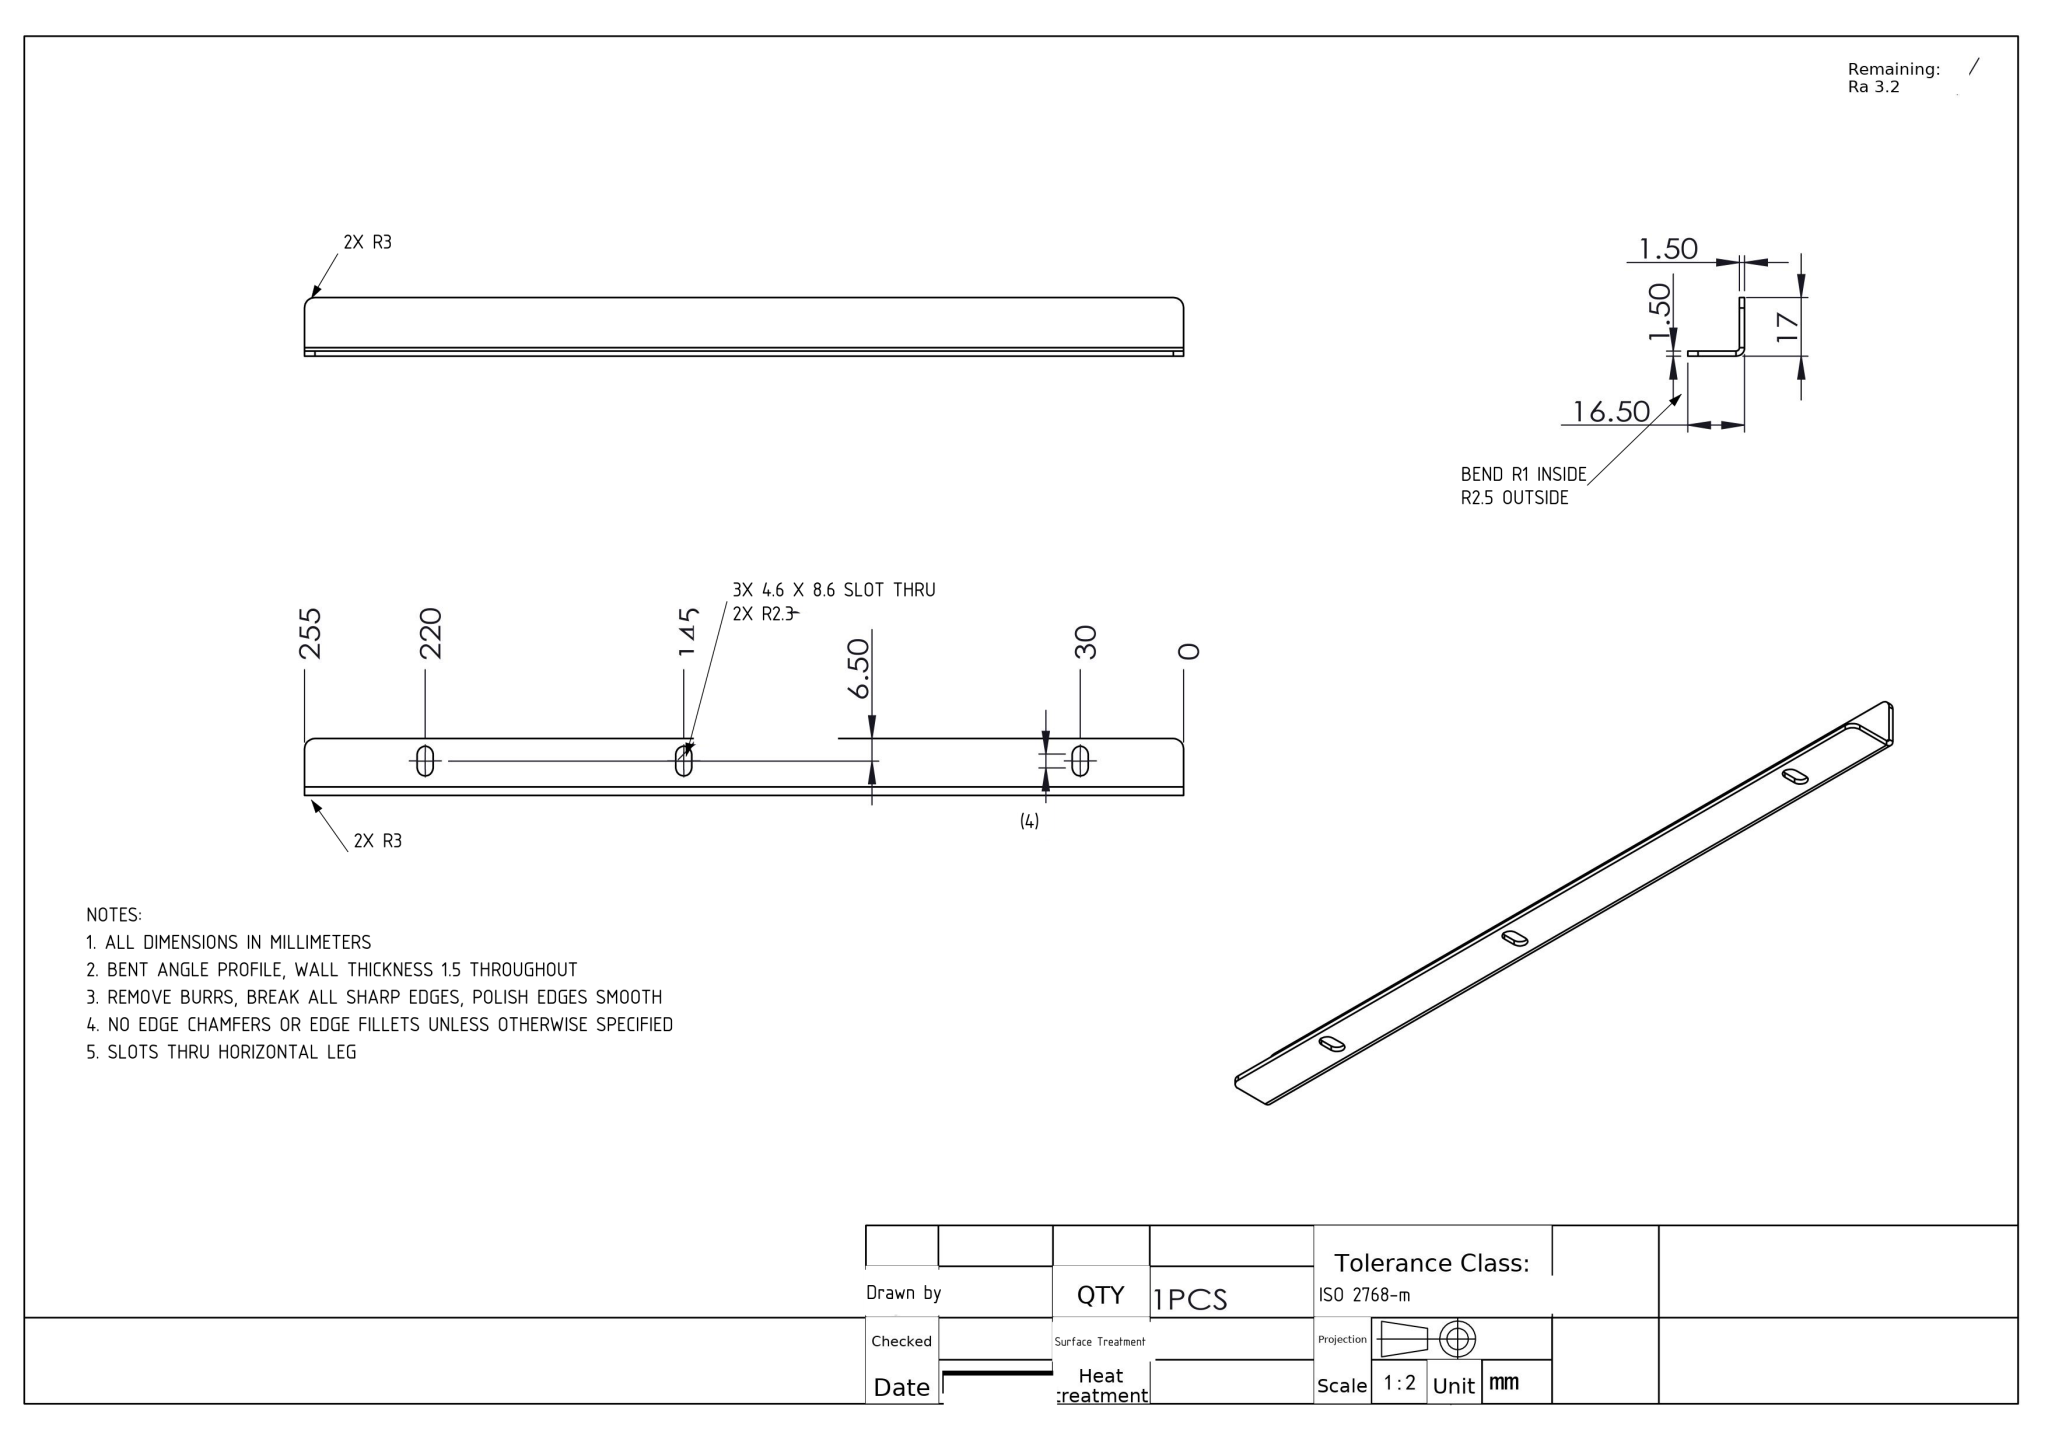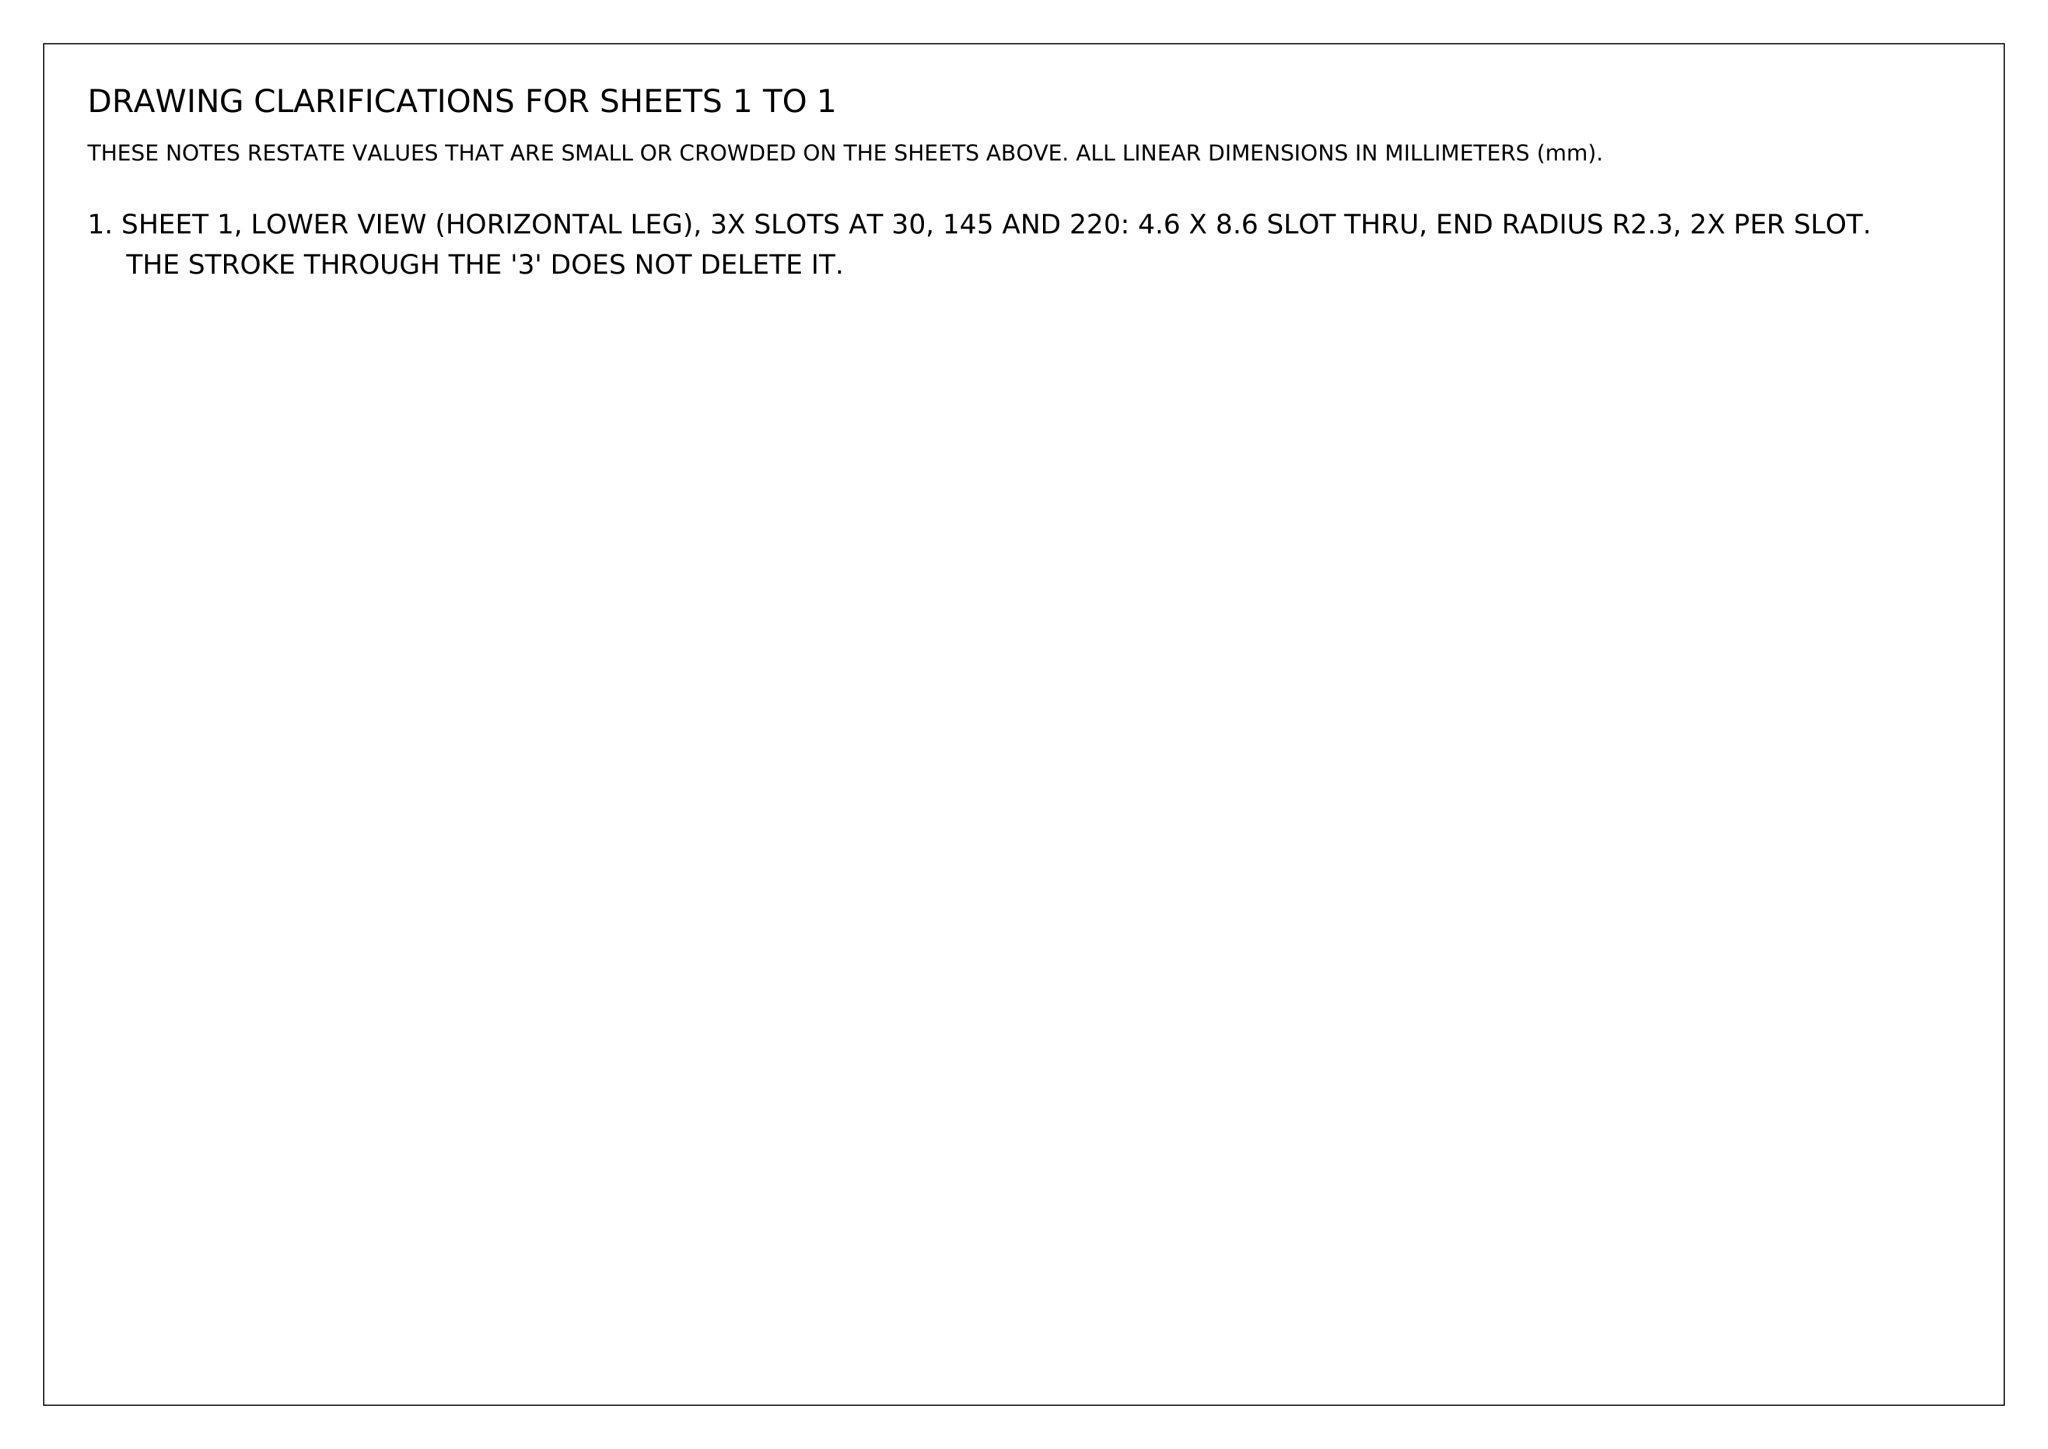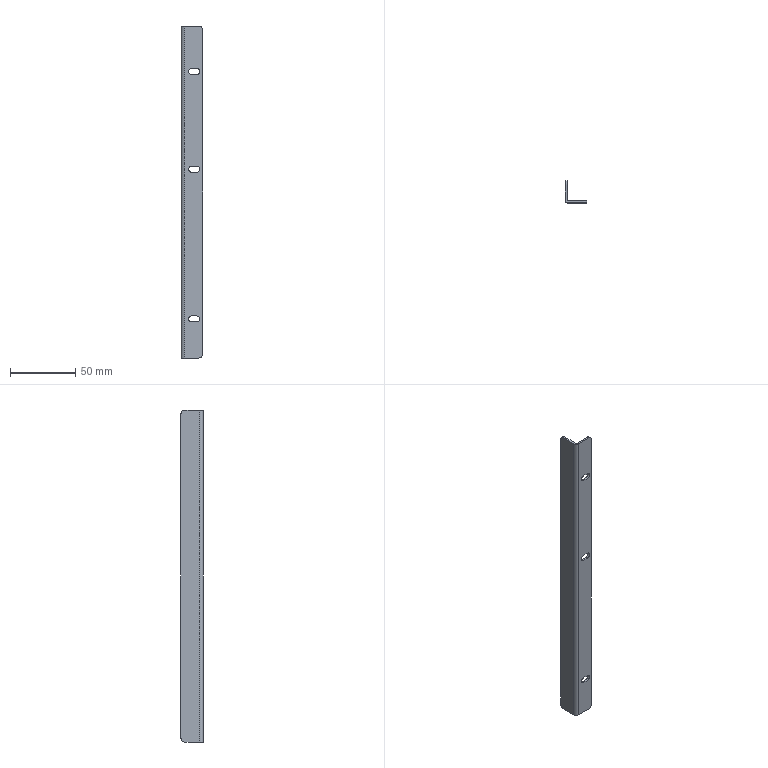Part | NX | mm | 1 solid | 30 faces | box 16.5 x 17 x 255 mm | volume 11784 mm3 | plane 18 | cylinder 12 | commonest cylinder face diameters 4.6 x6 6 x4 2 x1 5 x1